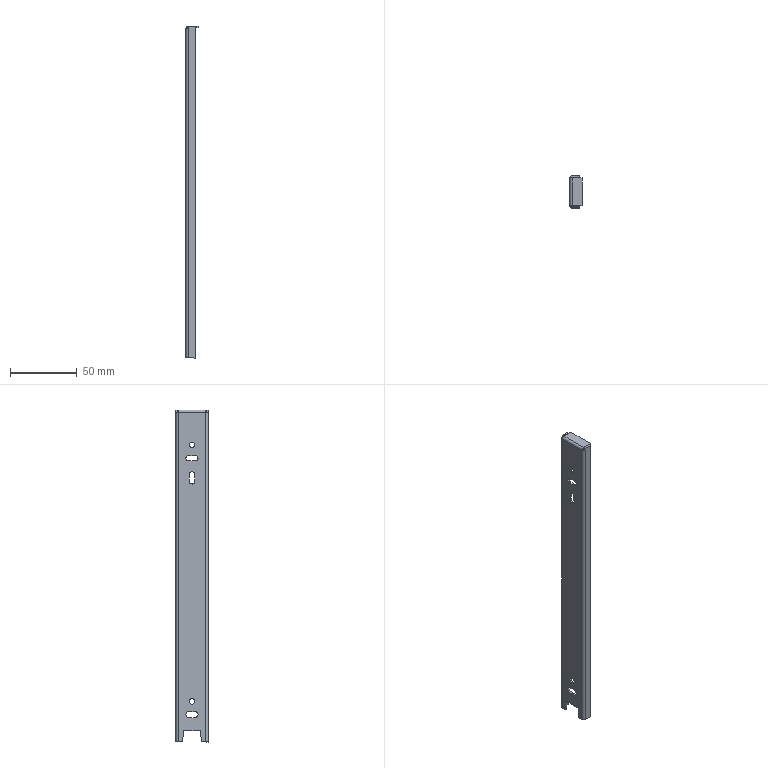Component | SolidWorks | PC-CAJ-P09-1_PC-CAJ-P14-1_Corredera C 250-1 | 1 solid | 49 faces | volume 10198 mm3 | plane 30 | cylinder 19 | commonest cylinder face diameters 4 x8 4.4 x5 1 x3 3.4 x3 | material Plain Carbon Steel